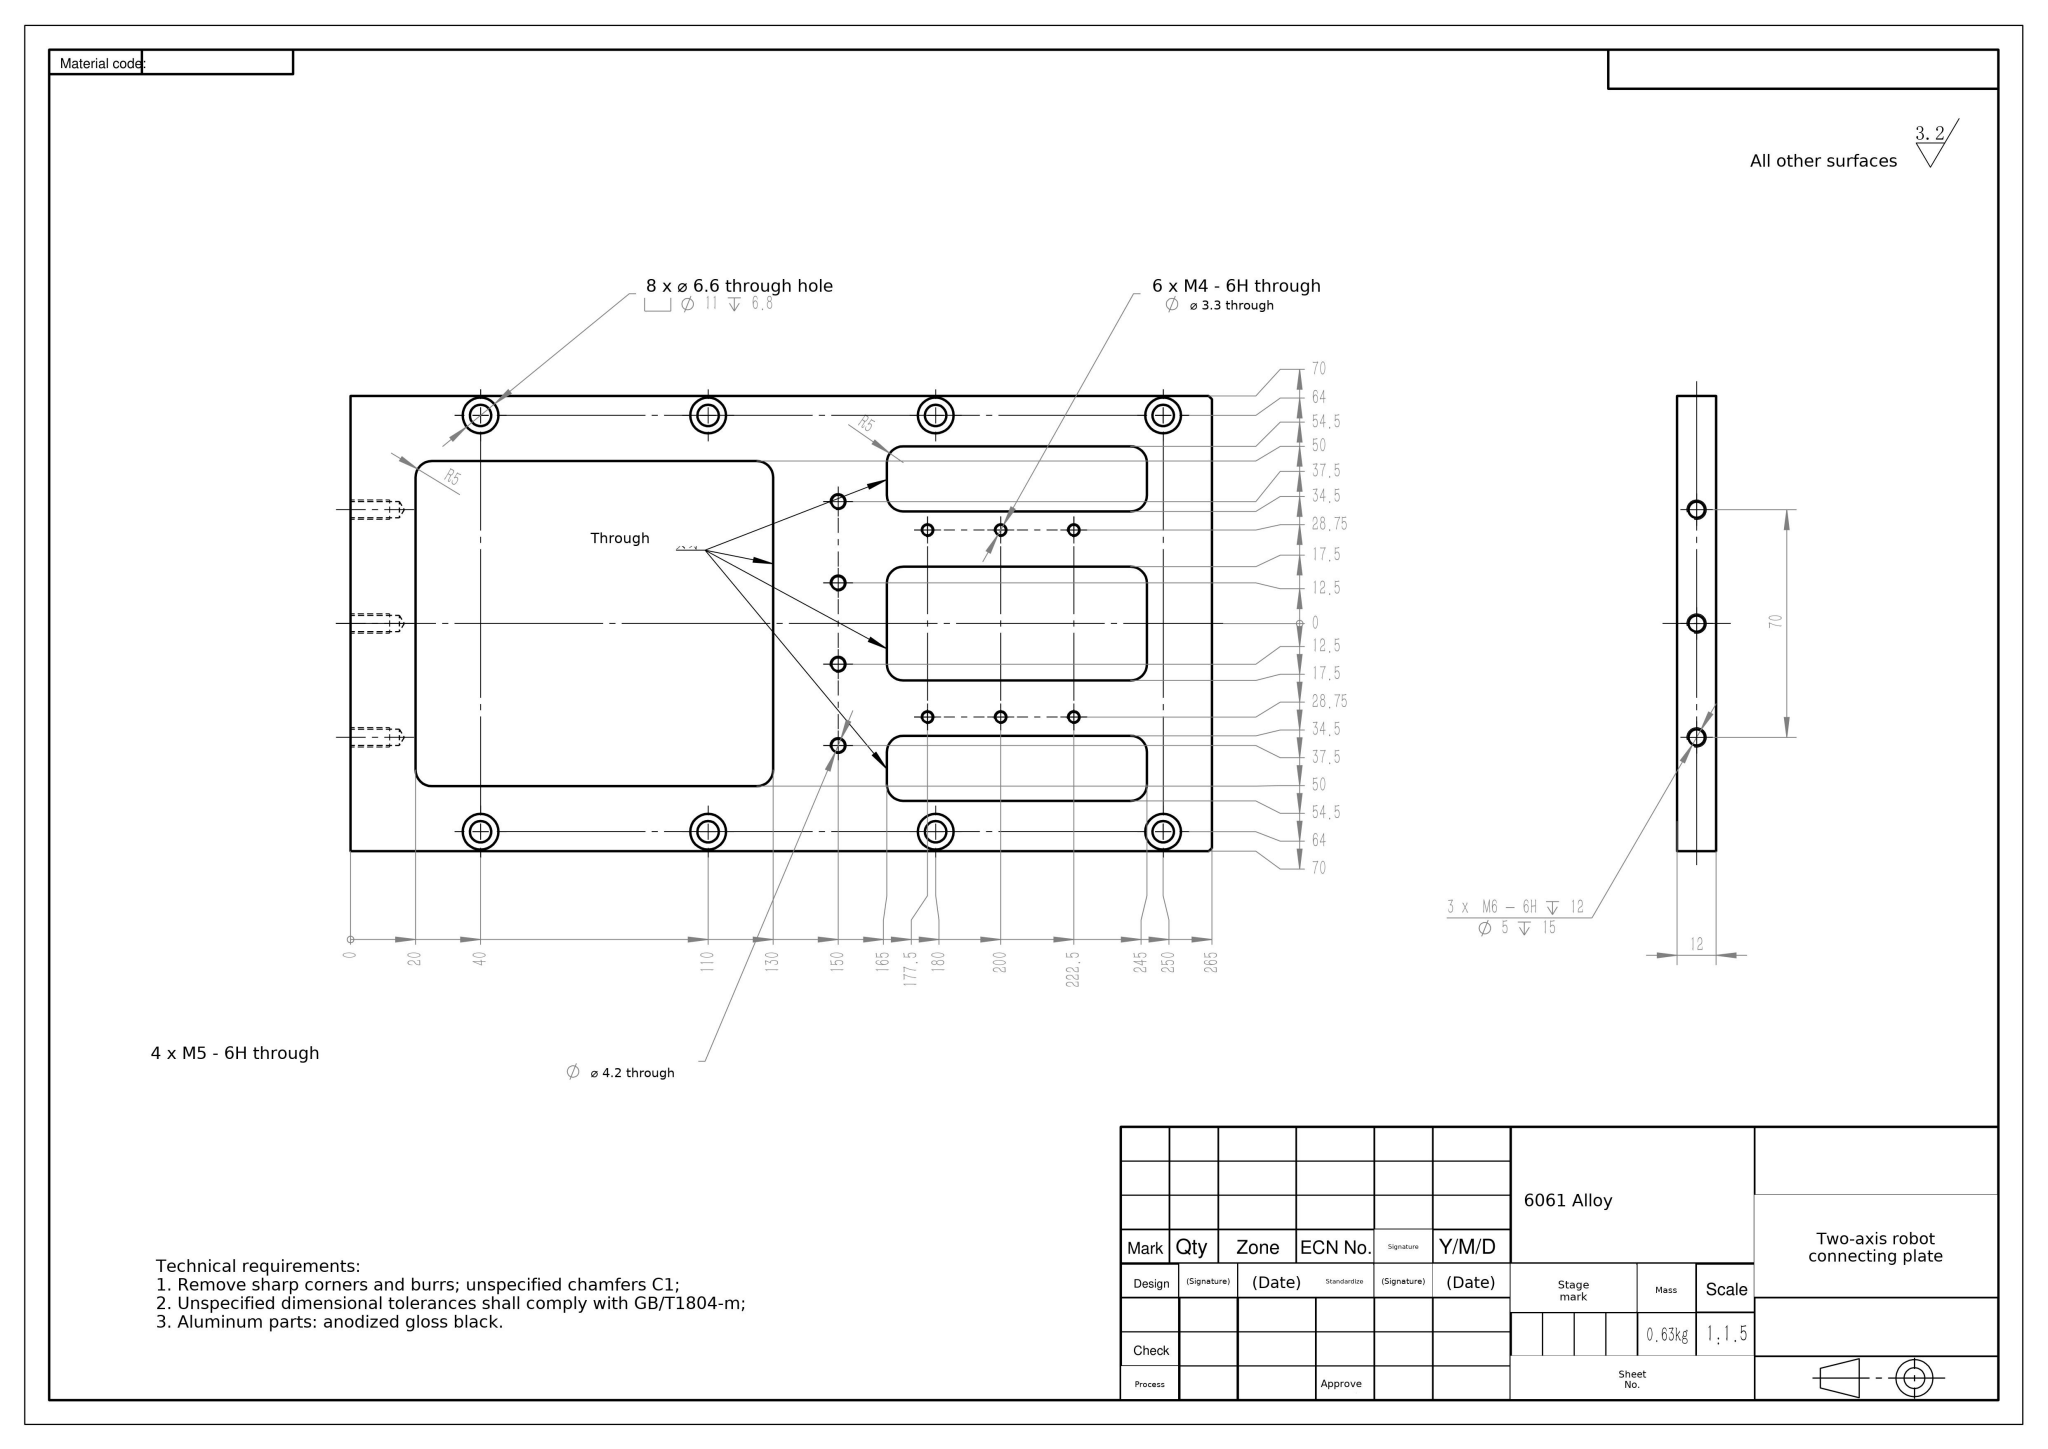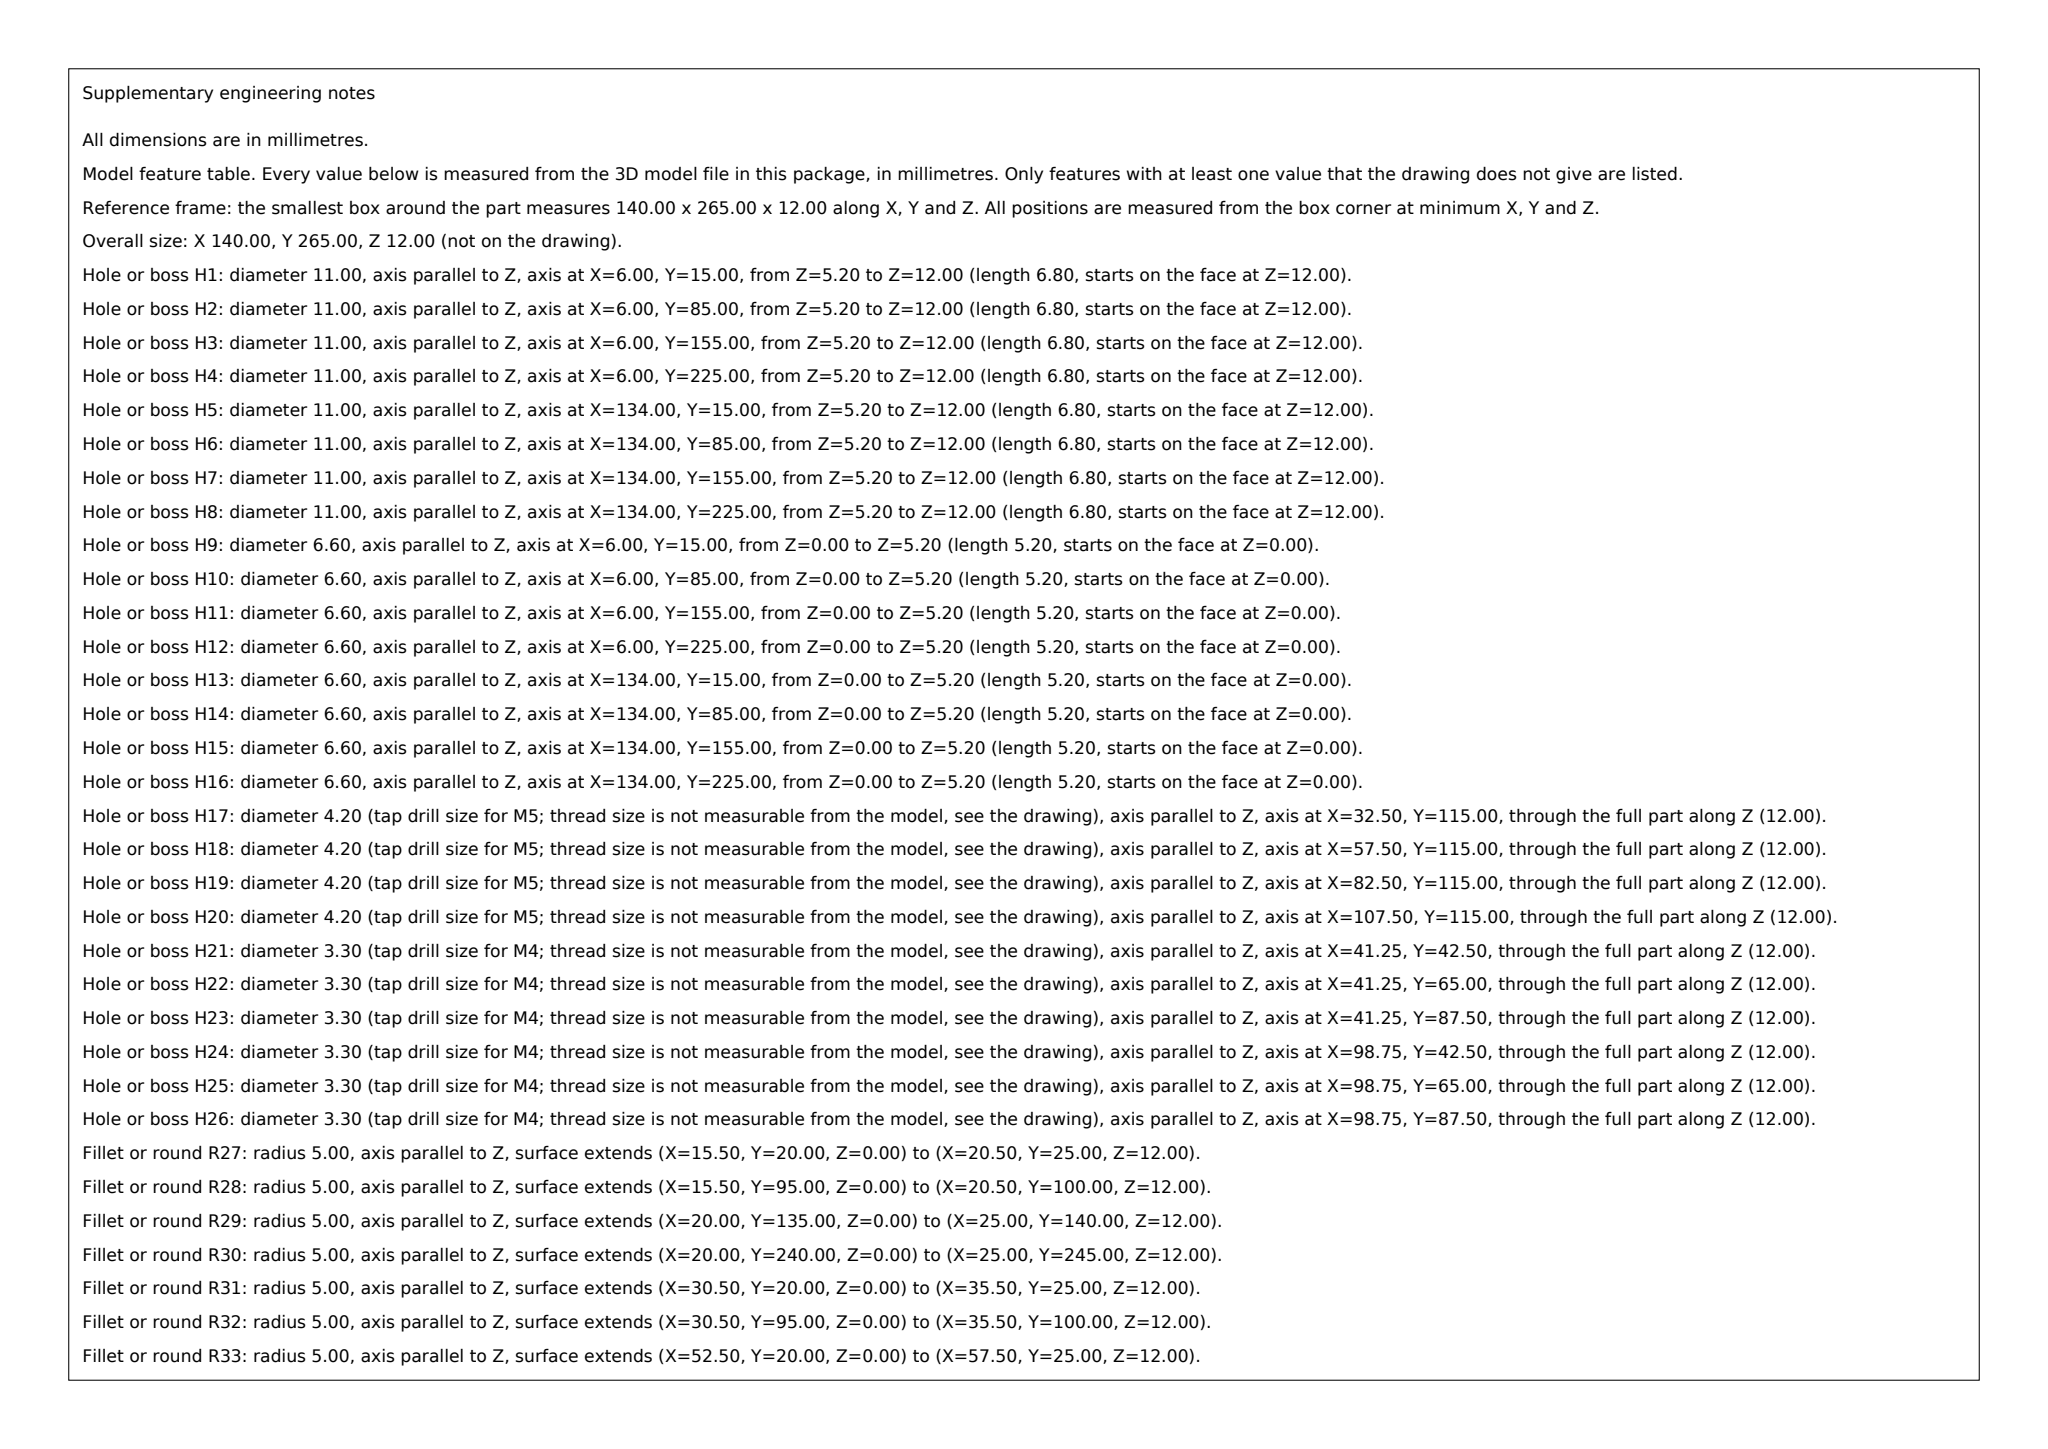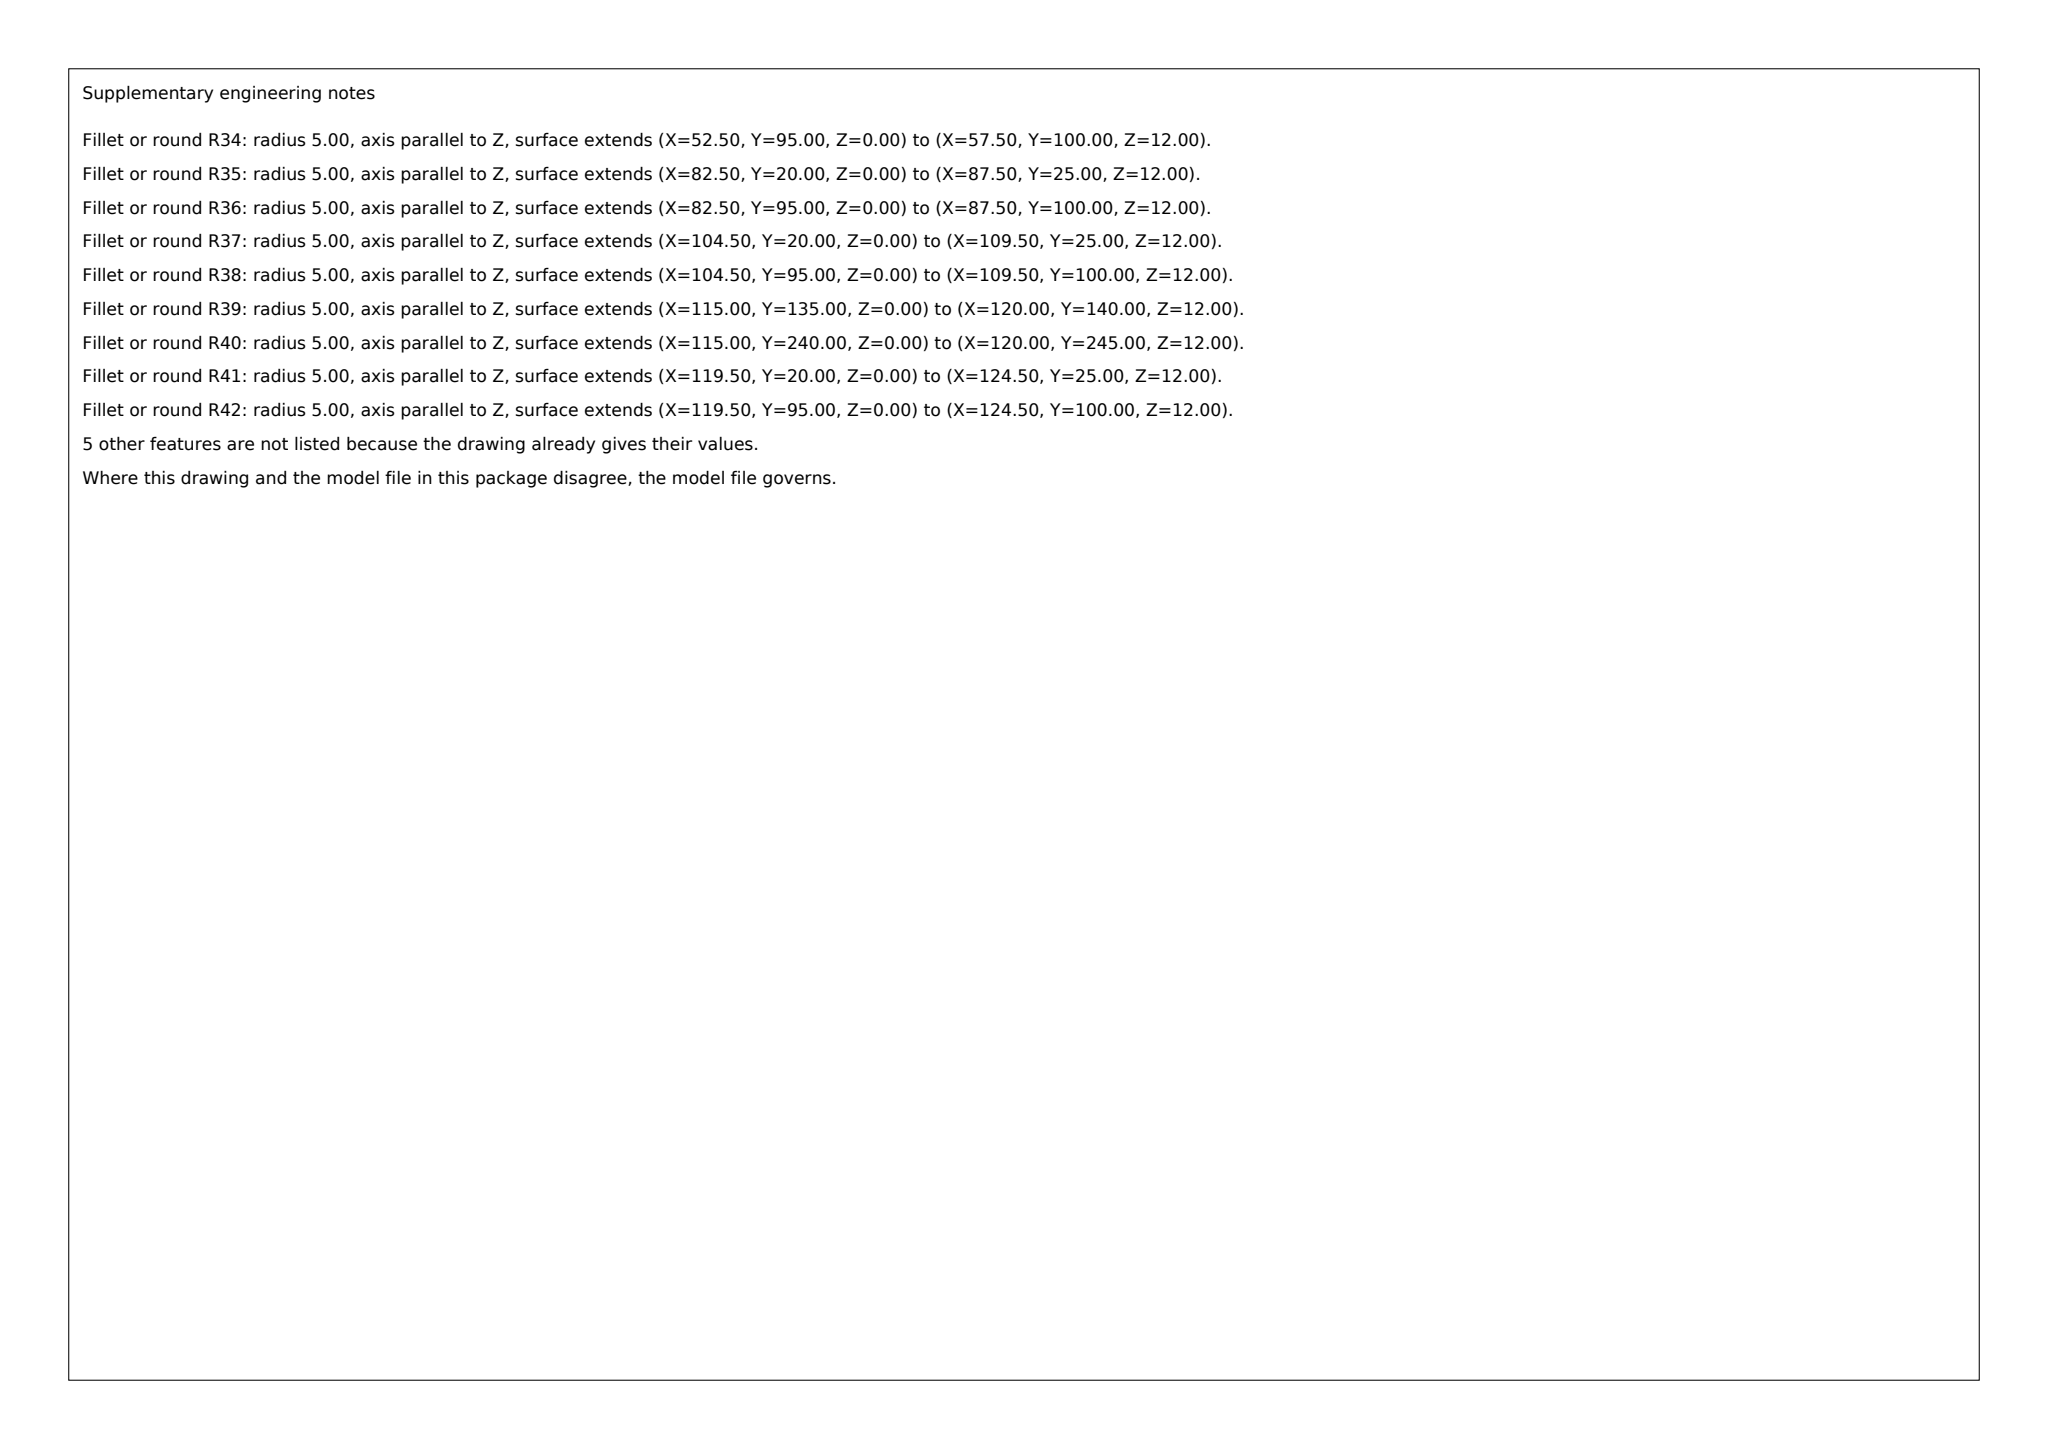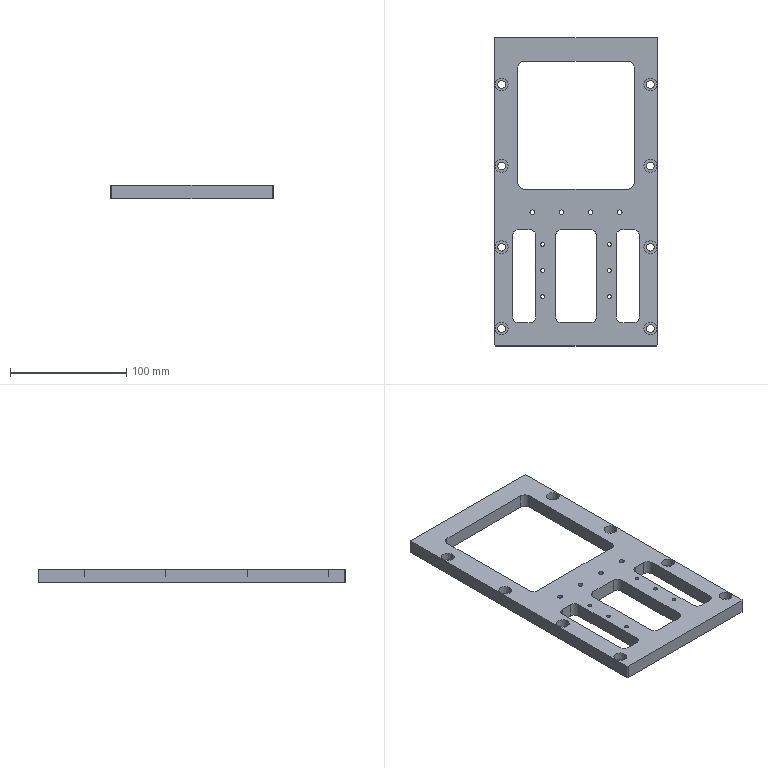Part | SolidWorks | mm | material 6061 Alloy | 1 solid | 112 faces | box 140 x 265 x 12 mm | volume 233431 mm3 | cylinder 74 | plane 32 | cone 6 | commonest cylinder face diameters 11 x16 6.6 x16 10 x16 3.3 x12 4.2 x8 5 x6
build123d program:
from build123d import *

# Parameters (mm, degrees)
SKETCH1_W                                         = 140
SKETCH1_H                                         = 265
BOSS_EXTRUDE1_DEPTH                               = 12
CUT_EXTRUDE1_DEPTH                                = 151.334
HOLE_SIZE_ACCORDING_TO_HEXAGON_SOCKET_D           = 6.6
HOLE_SIZE_ACCORDING_TO_HEXAGON_SOCKET_CBORE_D     = 11
HOLE_SIZE_ACCORDING_TO_HEXAGON_SOCKET_CBORE_DEPTH = 6.8
M6_TAPPED_HOLE1_D                                 = 5
M6_TAPPED_HOLE1_DEPTH                             = 15
M6_TAPPED_HOLE1_TIP                               = 1.502
M5_TAPPED_HOLE1_D                                 = 4.2
M4_TAPPED_HOLE1_D                                 = 3.3
CUT_EXTRUDE2_DEPTH                                = 151.334
CHAMFER1_SIZE                                     = 1


with BuildPart() as part:
    # Sketch1 → Boss-Extrude1 (new body)
    with BuildSketch(Plane.XY):
        Rectangle(SKETCH1_W, SKETCH1_H)
    extrude(amount=BOSS_EXTRUDE1_DEPTH)

    # Sketch2 → Cut-Extrude1 (cut, through all)
    with BuildSketch(Plane.XY.offset(12)):
        with BuildLine():
            Line((-45, 112.5), (45, 112.5))
            ThreePointArc((45, 112.5), (48.536, 111.036), (50, 107.5))
            Line((50, 107.5), (50, 7.5))
            ThreePointArc((50, 7.5), (48.536, 3.964), (45, 2.5))
            Line((45, 2.5), (-45, 2.5))
            ThreePointArc((-45, 2.5), (-48.536, 3.964), (-50, 7.5))
            Line((-50, 7.5), (-50, 107.5))
            ThreePointArc((-50, 107.5), (-48.536, 111.036), (-45, 112.5))
        make_face()
    extrude(amount=-CUT_EXTRUDE1_DEPTH, mode=Mode.SUBTRACT)

    # Hole Size _according to_ Hexagon Socket (through all)
    with Locations(Plane.XY.offset(12)):
        with Locations((-64, 92.5), (-64, 22.5), (-64, -47.5), (-64, -117.5), (64, -117.5), (64, -47.5), (64, 22.5), (64, 92.5)):
            CounterBoreHole(HOLE_SIZE_ACCORDING_TO_HEXAGON_SOCKET_D / 2, HOLE_SIZE_ACCORDING_TO_HEXAGON_SOCKET_CBORE_D / 2, HOLE_SIZE_ACCORDING_TO_HEXAGON_SOCKET_CBORE_DEPTH)

    # M6 Tapped Hole1
    with Locations(Plane(origin=(0, 132.5, 0), x_dir=(1, 0, 0), z_dir=(0, 1, 0))):
        with Locations((0, -6), (-35, -6), (35, -6)):
            Hole(M6_TAPPED_HOLE1_D / 2, depth=M6_TAPPED_HOLE1_DEPTH)
            with Locations((0, 0, -(M6_TAPPED_HOLE1_DEPTH + M6_TAPPED_HOLE1_TIP / 2))):  # 118° drill point
                Cone(0, M6_TAPPED_HOLE1_D / 2, M6_TAPPED_HOLE1_TIP, mode=Mode.SUBTRACT)

    # M5 Tapped Hole1 (through all)
    with Locations(Plane.XY.offset(12)):
        with Locations((-37.5, -17.5), (-12.5, -17.5), (12.5, -17.5), (37.5, -17.5)):
            Hole(M5_TAPPED_HOLE1_D / 2)

    # M4 Tapped Hole1 (through all)
    with Locations(Plane.XY.offset(12)):
        with Locations((-28.75, -45), (-28.75, -67.5), (-28.75, -90), (28.75, -90), (28.75, -67.5), (28.75, -45)):
            Hole(M4_TAPPED_HOLE1_D / 2)

    # Sketch11 → Cut-Extrude2 (cut, through all)
    with BuildSketch(Plane.XY.offset(12)):
        with BuildLine():
            Line((34.5, -37.5), (34.5, -107.5))
            ThreePointArc((34.5, -107.5), (35.964, -111.036), (39.5, -112.5))
            Line((39.5, -112.5), (49.5, -112.5))
            ThreePointArc((49.5, -112.5), (53.036, -111.036), (54.5, -107.5))
            Line((54.5, -107.5), (54.5, -37.5))
            ThreePointArc((54.5, -37.5), (53.036, -33.964), (49.5, -32.5))
            Line((49.5, -32.5), (39.5, -32.5))
            ThreePointArc((39.5, -32.5), (35.964, -33.964), (34.5, -37.5))
        make_face()
        with BuildLine():
            Line((-12.5, -112.5), (12.5, -112.5))
            ThreePointArc((12.5, -112.5), (16.036, -111.036), (17.5, -107.5))
            Line((17.5, -107.5), (17.5, -37.5))
            ThreePointArc((17.5, -37.5), (16.036, -33.964), (12.5, -32.5))
            Line((12.5, -32.5), (-12.5, -32.5))
            ThreePointArc((-12.5, -32.5), (-16.036, -33.964), (-17.5, -37.5))
            Line((-17.5, -37.5), (-17.5, -107.5))
            ThreePointArc((-17.5, -107.5), (-16.036, -111.036), (-12.5, -112.5))
        make_face()
        with BuildLine():
            Line((-49.5, -32.5), (-39.5, -32.5))
            ThreePointArc((-39.5, -32.5), (-35.964, -33.964), (-34.5, -37.5))
            Line((-34.5, -37.5), (-34.5, -107.5))
            ThreePointArc((-34.5, -107.5), (-35.964, -111.036), (-39.5, -112.5))
            Line((-39.5, -112.5), (-49.5, -112.5))
            ThreePointArc((-49.5, -112.5), (-53.036, -111.036), (-54.5, -107.5))
            Line((-54.5, -107.5), (-54.5, -37.5))
            ThreePointArc((-54.5, -37.5), (-53.036, -33.964), (-49.5, -32.5))
        make_face()
    extrude(amount=-CUT_EXTRUDE2_DEPTH, mode=Mode.SUBTRACT)

    # Chamfer1
    chamfer1_edges = [part.edges().sort_by_distance(p)[0] for p in [
        (70, -132.5, 6),
        (-70, -132.5, 6),
    ]]
    chamfer(chamfer1_edges, length=CHAMFER1_SIZE)


solid = part.part